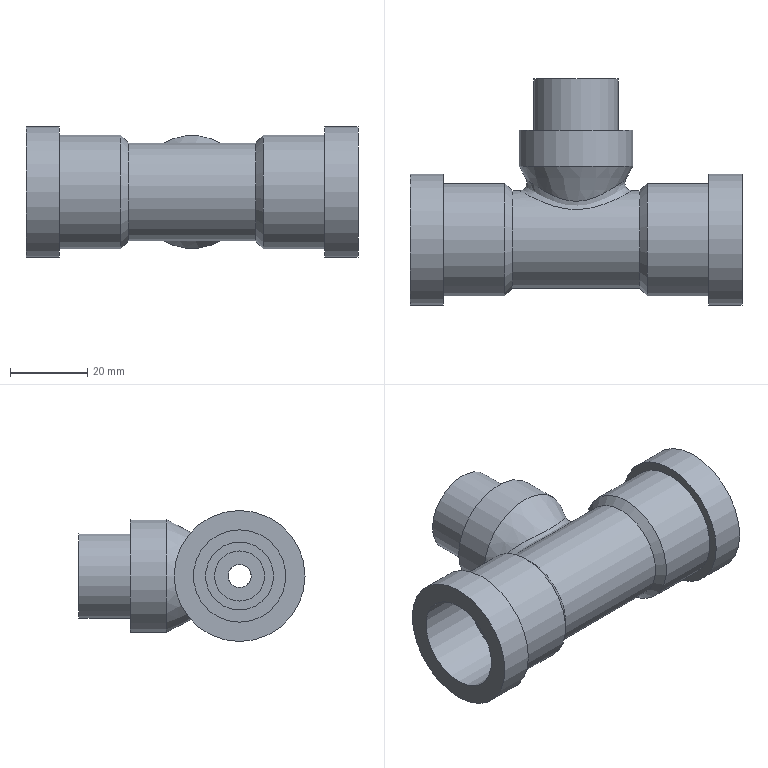Component | NX | CHECK_VALVE | 1 solid | 37 faces | volume 41433 mm3 | cylinder 18 | plane 14 | cone 4 | spline 1 | commonest cylinder face diameters 29.4 x3 6 x2 34 x2 24 x2 17.6 x2 13 x2 25.4 x1 14.6 x1